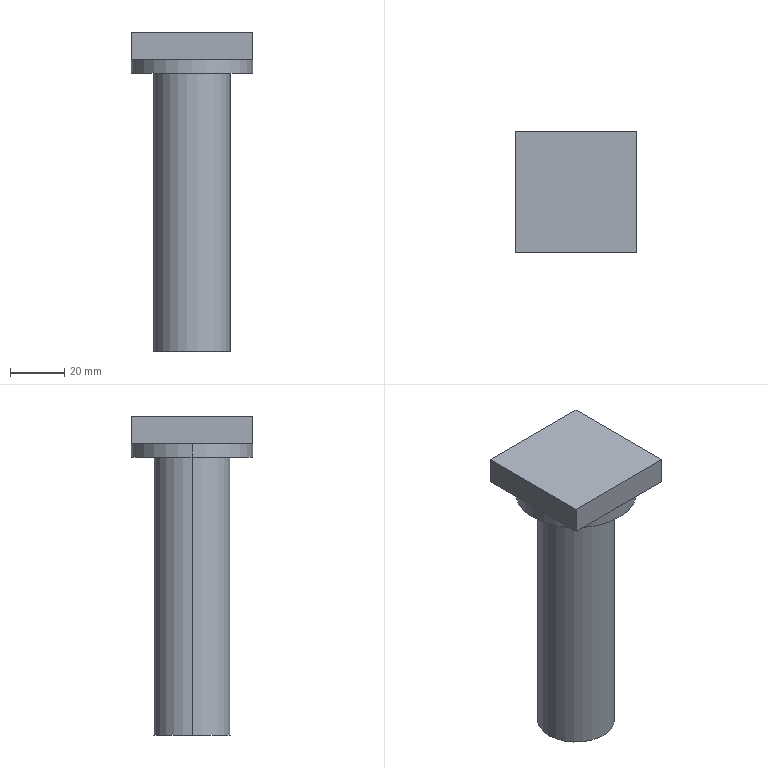CAM job | Mastercam | mm | 13 operations | part box 72 x 55 x 118
1. Contour (Ramp) | 3 - 3 平铣刀
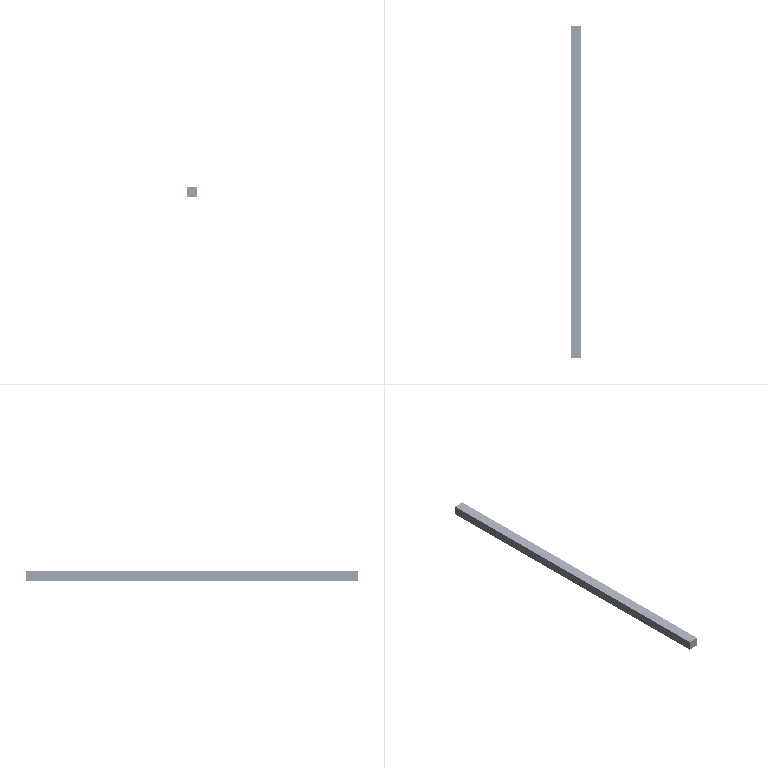2. Contour (Ramp) | 3 - 3 平铣刀
3. Contour (2D chamfer) | 5 - 4 倒角刀
4. Facing | 20 - 63 平铣刀
5. Contour (Ramp) | 9 - 10 平铣刀
6. Contour (2D) | 10 - 10 平铣刀
7. Contour (2D chamfer) | 5 - 4 倒角刀
8. Facing | 20 - 63 平铣刀
9. 2D High Speed (2D Area Mill) | 8 - 8 平铣刀
10. 2D High Speed (2D Area Mill) | 8 - 8 平铣刀
11. Contour (2D) | 8 - 8 平铣刀
12. Contour (2D chamfer) | 5 - 4 倒角刀
13. Drill/Counterbore | 5 - 4 倒角刀